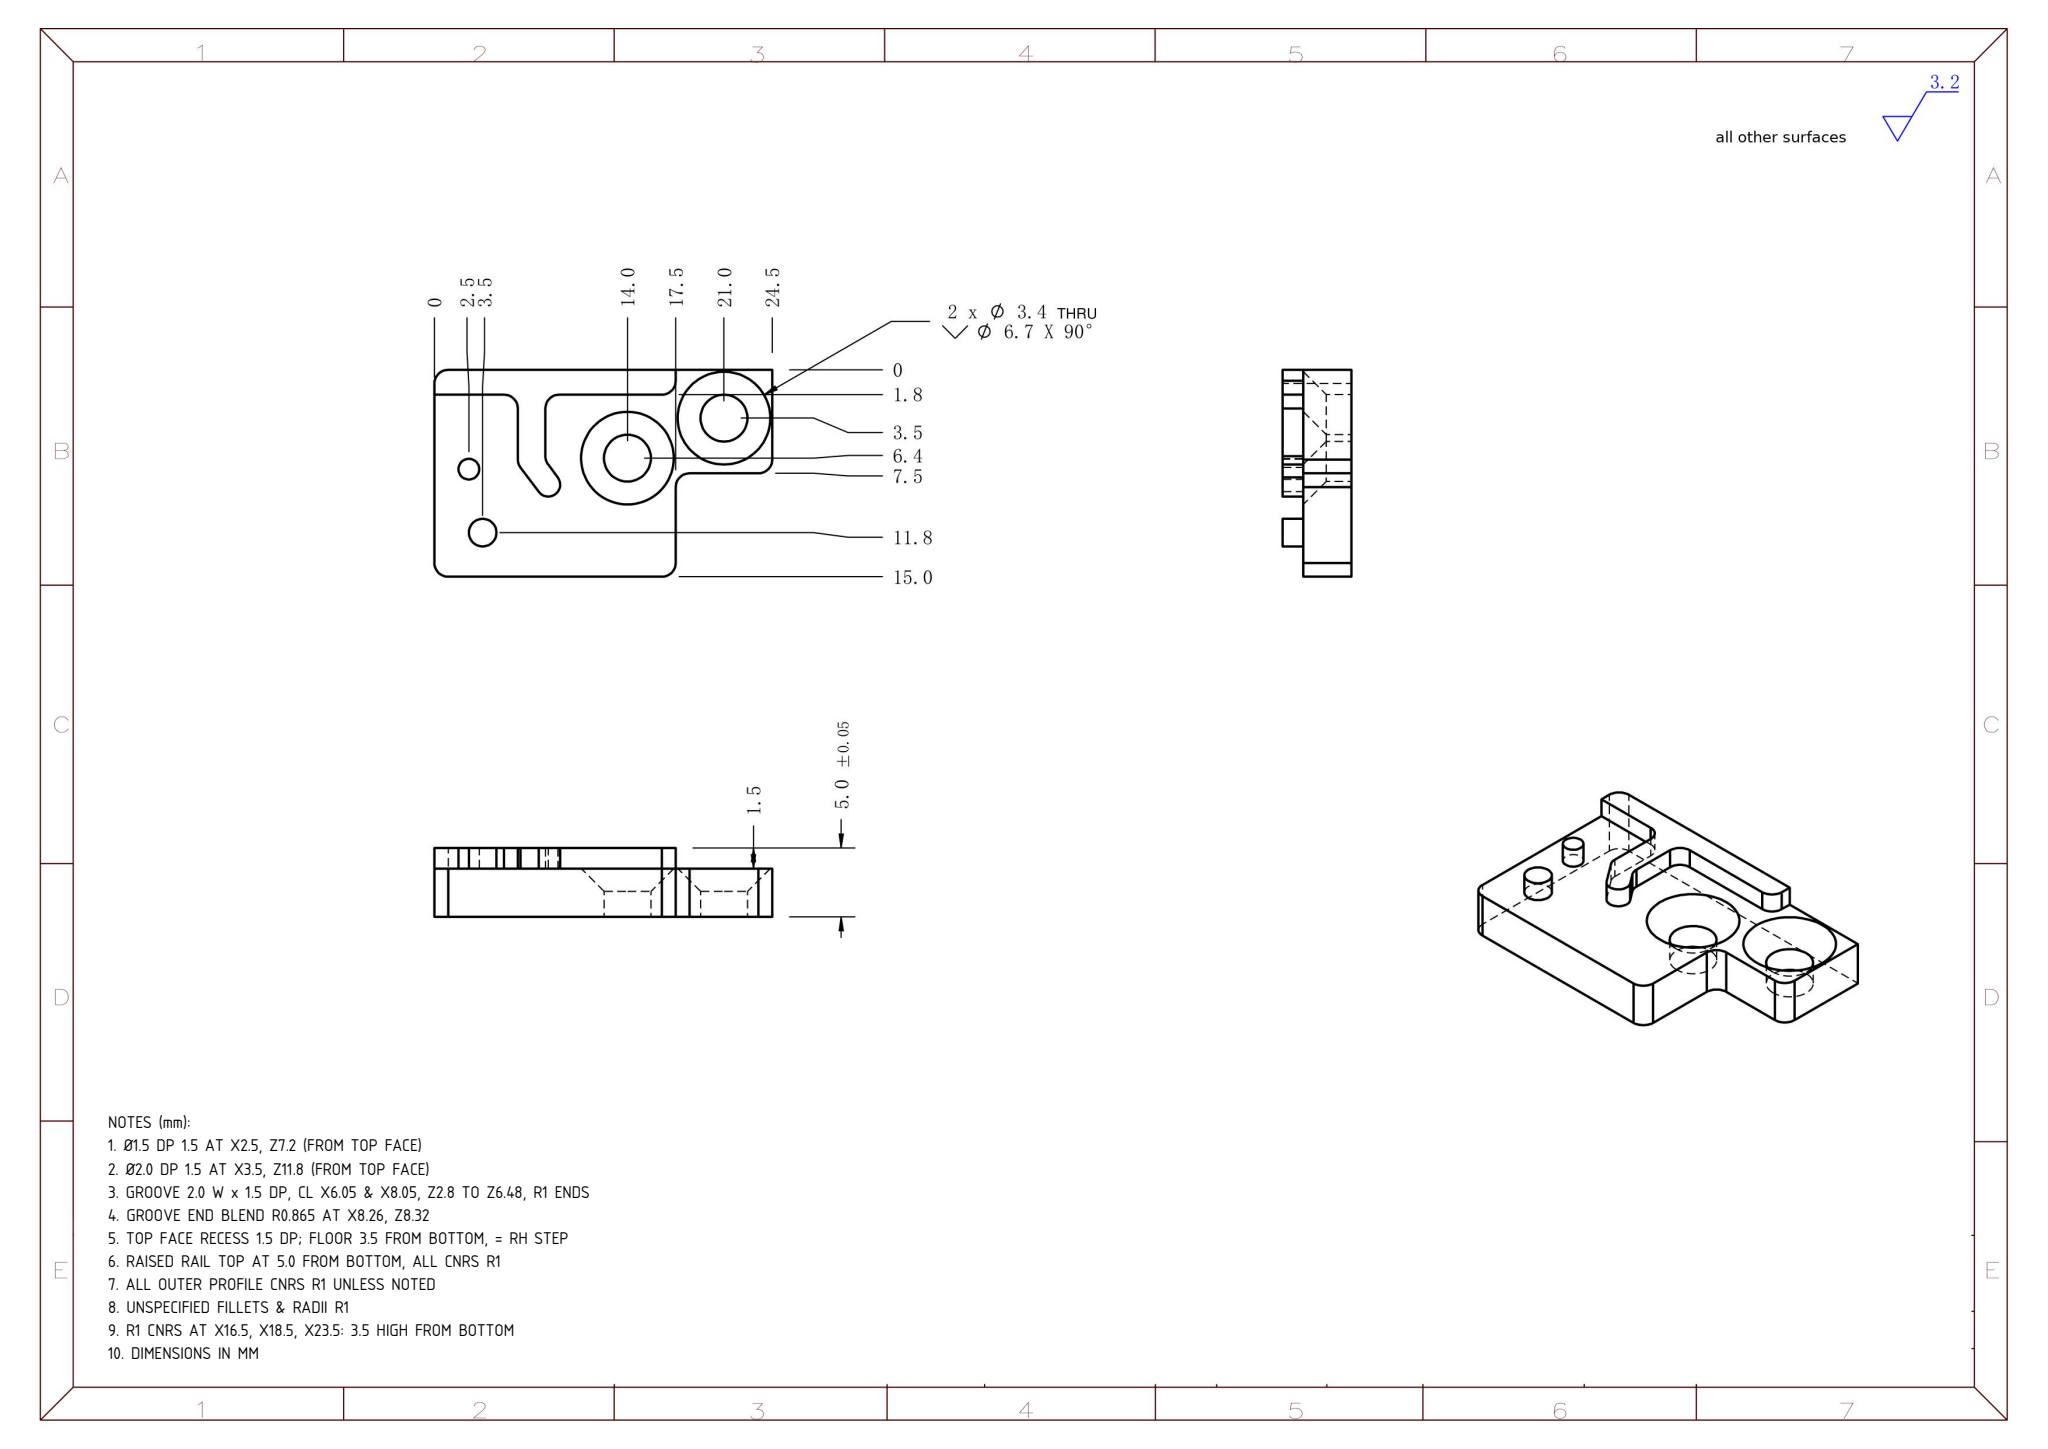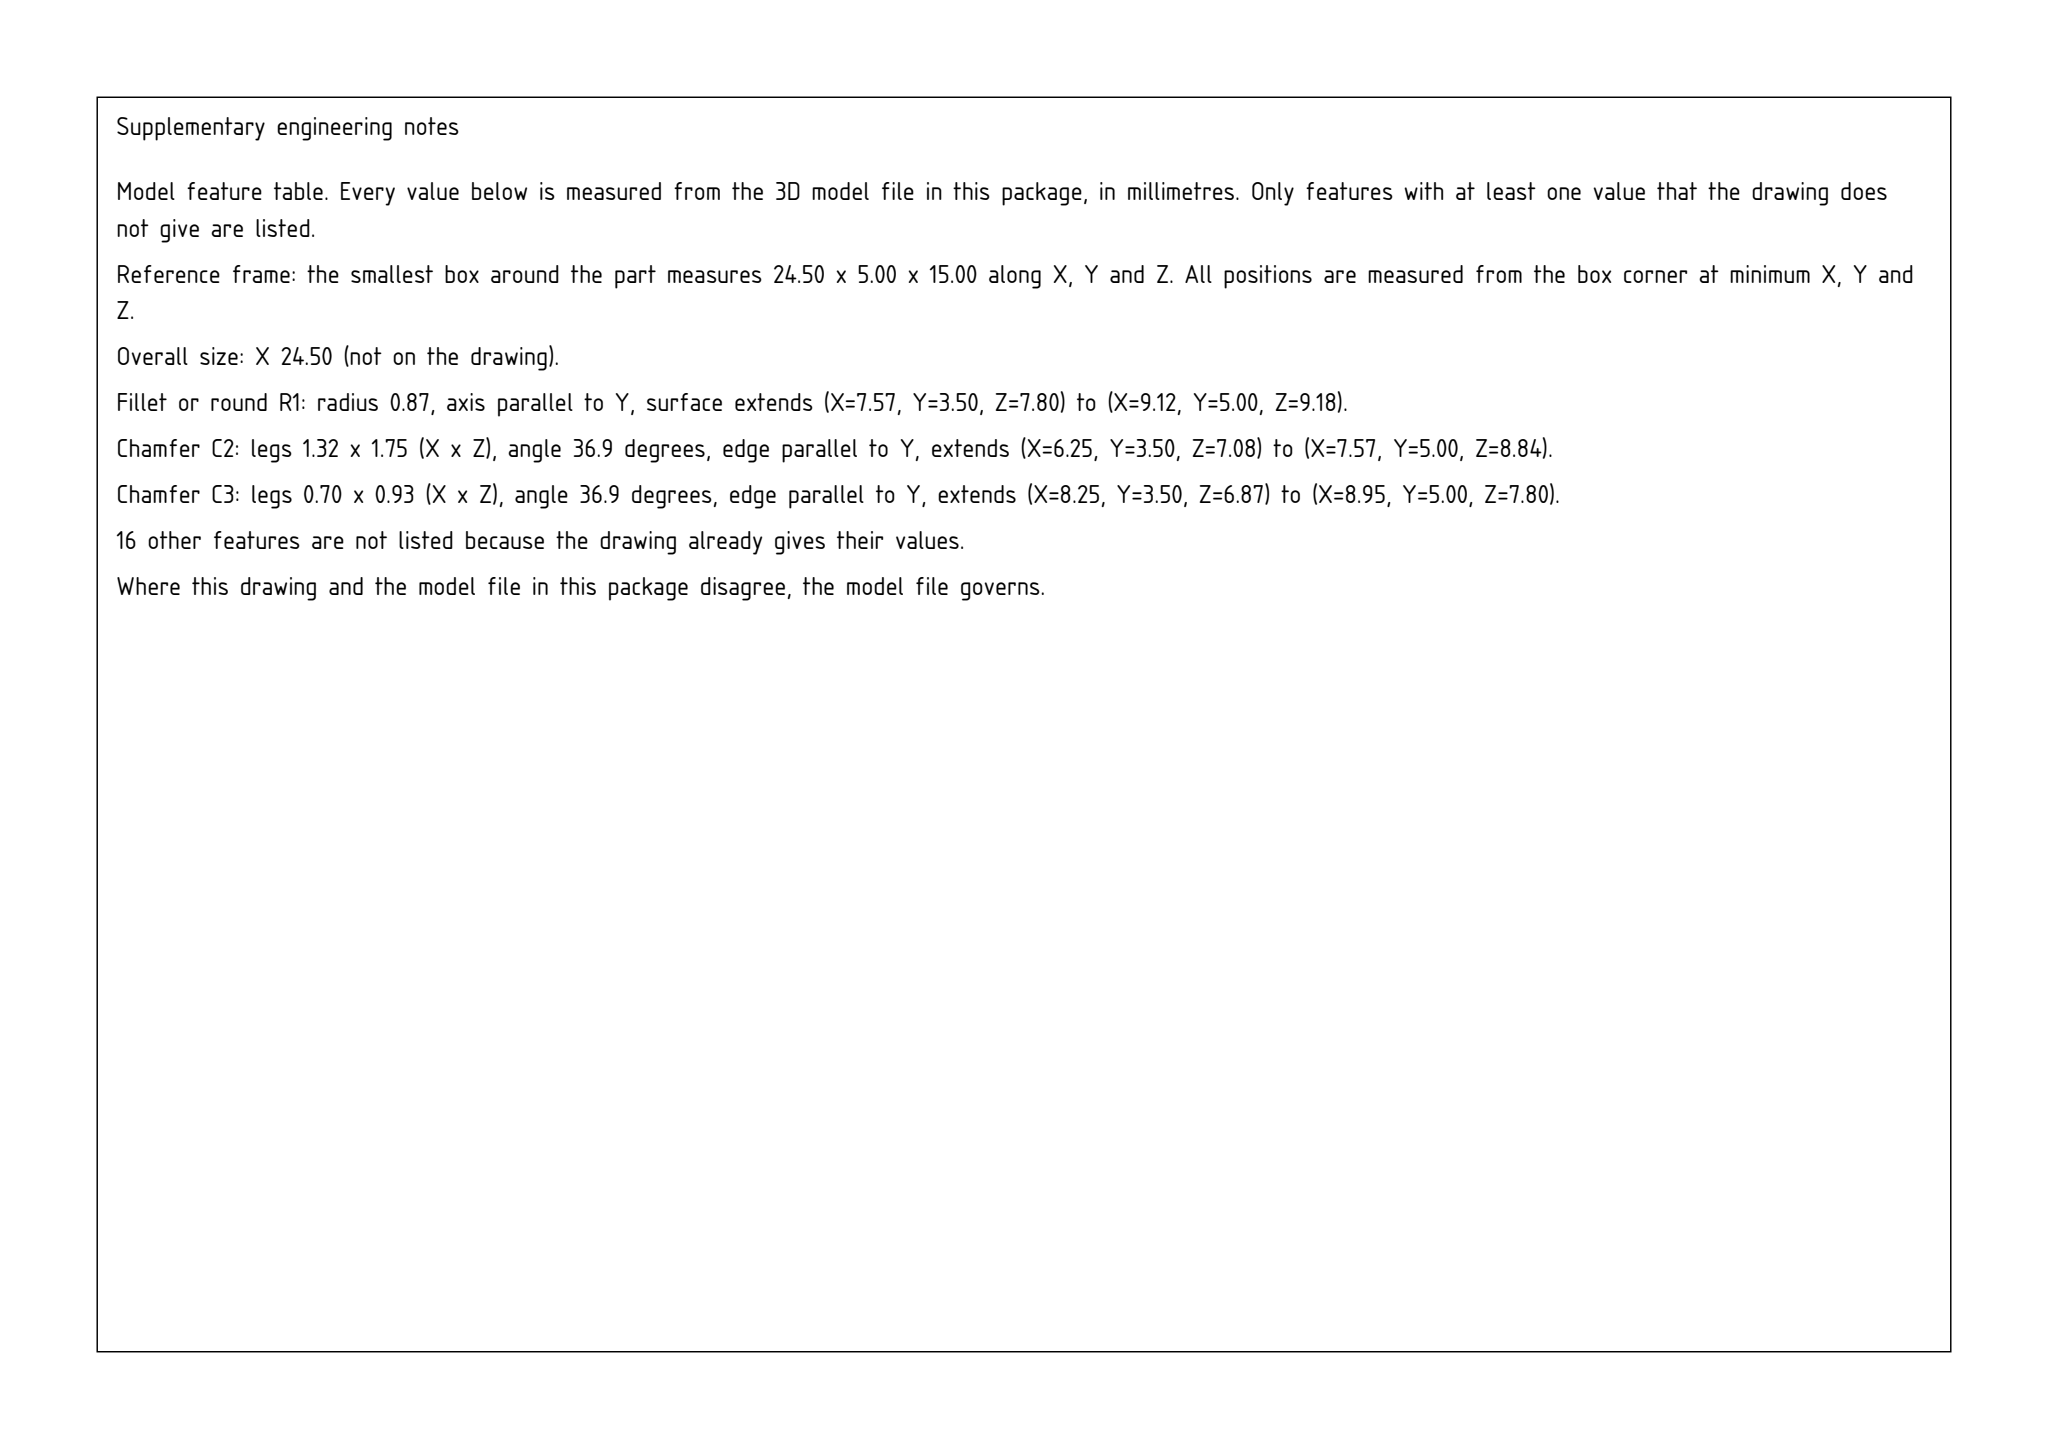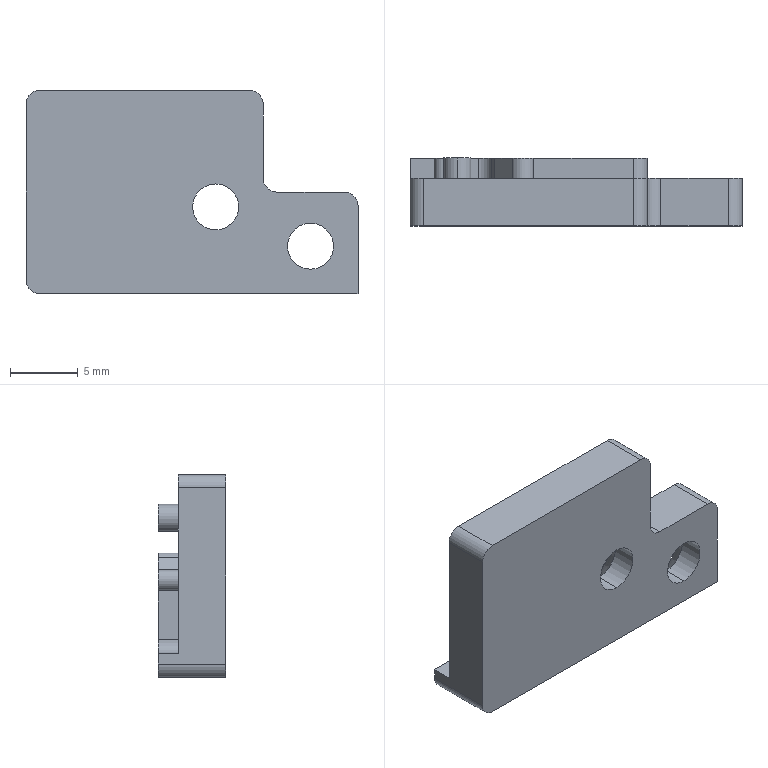Part | SolidWorks | mm | 1 solid | 41 faces | box 24.5 x 5 x 15 mm | volume 1074 mm3 | cylinder 19 | plane 18 | cone 4 | commonest cylinder face diameters 2 x12 3.4 x4 1.5 x2 1.73 x1
Drawing notes:
Ø1.5 DP 1.5 AT X2.5, Z7.2 (FROM TOP FACE) | from the solid: cyl dia 1.5, axis y, pos (2.5,-,7.2), len 1.5
Ø2.0 DP 1.5 AT X3.5, Z11.8 (FROM TOP FACE) | from the solid: cyl dia 2.0, axis y, pos (3.5,-,11.8), len 1.5
GROOVE 2.0 W x 1.5 DP, CL X6.05 & X8.05, Z2.8 TO Z6.48, R1 ENDS | from the solid: 2.0 dia y-cyls len 1.5 at (5.05,2.8)(7.05,6.48)(9.05,2.8)(9.05,6.27); x planes 6.05 & 8.05
GROOVE END BLEND R0.865 AT X8.26, Z8.32 | from the solid: cyl dia 1.73, axis y, pos (8.26,-,8.32), len 1.5
TOP FACE RECESS 1.5 DP; FLOOR 3.5 FROM BOTTOM, = RH STEP | from the solid: y planes 0.0, 3.5, 5.0; section 5.0 OAL w/ 1.5 step
RAISED RAIL TOP AT 5.0 FROM BOTTOM, ALL CNRS R1 | from the solid: y=5.0 faces (3); 2.0 dia corner cyls
ALL OUTER PROFILE CNRS R1 UNLESS NOTED | from the solid: 2.0 dia y-cyls at (1.0,1.0) len 5.0, (1.0,14.0), (16.5,0.8), (16.5,14.0)
UNSPECIFIED FILLETS & RADII R1 | from the solid: all corner cyls dia 2.0 = R1; no other fillet radii in model
R1 CNRS AT X16.5, X18.5, X23.5: 3.5 HIGH FROM BOTTOM | from the solid: 2.0 dia y-cyls len 3.5 at (16.5,14.0)(18.5,8.5)(23.5,6.5)
DIMENSIONS IN MM | from the solid: bbox 24.5 x 5.0 x 15.0 mm
build123d program:
from build123d import *

# Parameters (mm, degrees)
SKETCH1_W                                            = 24.5
SKETCH1_H                                            = 15
BOSS_EXTRUDE1_DEPTH                                  = 5
SKETCH2_R                                            = 0.75
SKETCH2_R_2                                          = 1
CUT_EXTRUDE1_DEPTH                                   = 1.5
CUT_EXTRUDE2_REACH                                   = 17.209
SKETCH5_W                                            = 7
SKETCH5_H                                            = 7.5
CUT_EXTRUDE3_DEPTH                                   = 10
FILLET1_R                                            = 1
M3_HEXAGON_COUNTERSUNK_HEAD_SCREW_COUNTE_D           = 3.4
M3_HEXAGON_COUNTERSUNK_HEAD_SCREW_COUNTE_CSINK_D     = 6.72
M3_HEXAGON_COUNTERSUNK_HEAD_SCREW_COUNTE_CSINK_ANGLE = 90


with BuildPart() as part:
    # Sketch1 → Boss-Extrude1 (new body)
    with BuildSketch(Plane(origin=(0, 0, 0), x_dir=(1, 0, 0), z_dir=(0, 1, 0))):
        Rectangle(SKETCH1_W, SKETCH1_H)
    extrude(amount=BOSS_EXTRUDE1_DEPTH)

    # Sketch2 → Cut-Extrude1 (cut)
    with BuildSketch(Plane(origin=(0, 5, 0), x_dir=(1, 0, 0), z_dir=(0, 1, 0))):
        with BuildLine():
            Line((5.25, 5.7), (5.25, 7.5))
            Line((5.25, 7.5), (12.25, 7.5))
            Line((12.25, 7.5), (12.25, -7.5))
            Line((12.25, -7.5), (-12.25, -7.5))
            Line((-12.25, -7.5), (-12.25, 5.7))
            Line((-12.25, 5.7), (-6.45, 5.7))
            Line((-6.45, 5.7), (-6.45, 0.6))
            Line((-6.45, 0.6), (-3.75, -3))
            Line((-3.75, -3), (-3.649, -4.844))
            ThreePointArc((-3.649, -4.844), (-2.598, -5.559), (-2.183, -4.358))
            Line((-2.183, -4.358), (-2.95, -3.2))
            Line((-2.95, -3.2), (-0.95, -1))
            Line((-0.95, -1), (-3.95, 1))
            Line((-3.95, 1), (-3.95, 5.7))
            Line((-3.95, 5.7), (5.25, 5.7))
        make_face()
        with Locations(Location((-9.75, 0.3, 0), (0, 0, 270))):
            Circle(SKETCH2_R, mode=Mode.SUBTRACT)
        with Locations(Location((-8.75, -4.3, 0), (0, 0, 270))):
            Circle(SKETCH2_R_2, mode=Mode.SUBTRACT)
    extrude(amount=-CUT_EXTRUDE1_DEPTH, mode=Mode.SUBTRACT)

    # Sketch5 → Cut-Extrude2 (cut, up to next)
    with BuildSketch(Plane(origin=(0, 5, 0), x_dir=(1, 0, 0), z_dir=(0, 1, 0)), mode=Mode.PRIVATE) as cut_extrude2_sk1:
        with Locations((8.75, -3.75)):
            Rectangle(SKETCH5_W, SKETCH5_H)
    cut_extrude2_tool1 = extrude(cut_extrude2_sk1.sketch, amount=-CUT_EXTRUDE2_REACH, mode=Mode.PRIVATE) & part.part
    add(cut_extrude2_tool1.solids().sort_by_distance((8.75, 5, 3.75))[0], mode=Mode.SUBTRACT)

    # Sketch6 → Cut-Extrude3 (cut)
    with BuildSketch(Plane(origin=(0, 3.5, 0), x_dir=(1, 0, 0), z_dir=(0, 1, 0))):
        with BuildLine():
            Line((-6.7, 5.7), (-6.2, 5.7))
            Line((-6.2, 5.7), (-6.2, 0.6833))
            Line((-6.2, 0.6833), (-4.684, -1.338))
            ThreePointArc((-4.684, -1.338), (-3.473, -1.511), (-3.3, -0.3))
            Line((-3.3, -0.3), (-4.2, 0.9))
            Line((-4.2, 0.9), (-4.2, 5.7))
            Line((-4.2, 5.7), (-0.95, 5.7))
            Line((-0.95, 5.7), (-0.95, -5.6))
            Line((-0.95, -5.6), (-6.7, -5.6))
            Line((-6.7, -5.6), (-6.7, 5.7))
        make_face()
    extrude(amount=CUT_EXTRUDE3_DEPTH, mode=Mode.SUBTRACT)

    # Fillet1
    fillet1_edges = [part.edges().sort_by_distance(p)[0] for p in [
        (-12.25, 1.75, 7.5),
        (5.25, 4.25, -5.7),
        (5.25, 1.75, 7.5),
        (5.25, 1.75, 0),
        (12.25, 1.75, 0),
        (-12.25, 2.5, -7.5),
        (-4.2, 4.25, -5.7),
        (-4.2, 4.25, -0.9),
        (-6.2, 4.25, -0.6833),
        (-6.2, 4.25, -5.7),
    ]]
    fillet(fillet1_edges, radius=FILLET1_R)

    # M3 Hexagon Countersunk Head Screw Counte (through all)
    with Locations(Plane(origin=(0, 3.5, 0), x_dir=(1, 0, 0), z_dir=(0, 1, 0))):
        with Locations((8.75, 4), (1.75, 1.1)):
            CounterSinkHole(M3_HEXAGON_COUNTERSUNK_HEAD_SCREW_COUNTE_D / 2, M3_HEXAGON_COUNTERSUNK_HEAD_SCREW_COUNTE_CSINK_D / 2, counter_sink_angle=M3_HEXAGON_COUNTERSUNK_HEAD_SCREW_COUNTE_CSINK_ANGLE)


solid = part.part